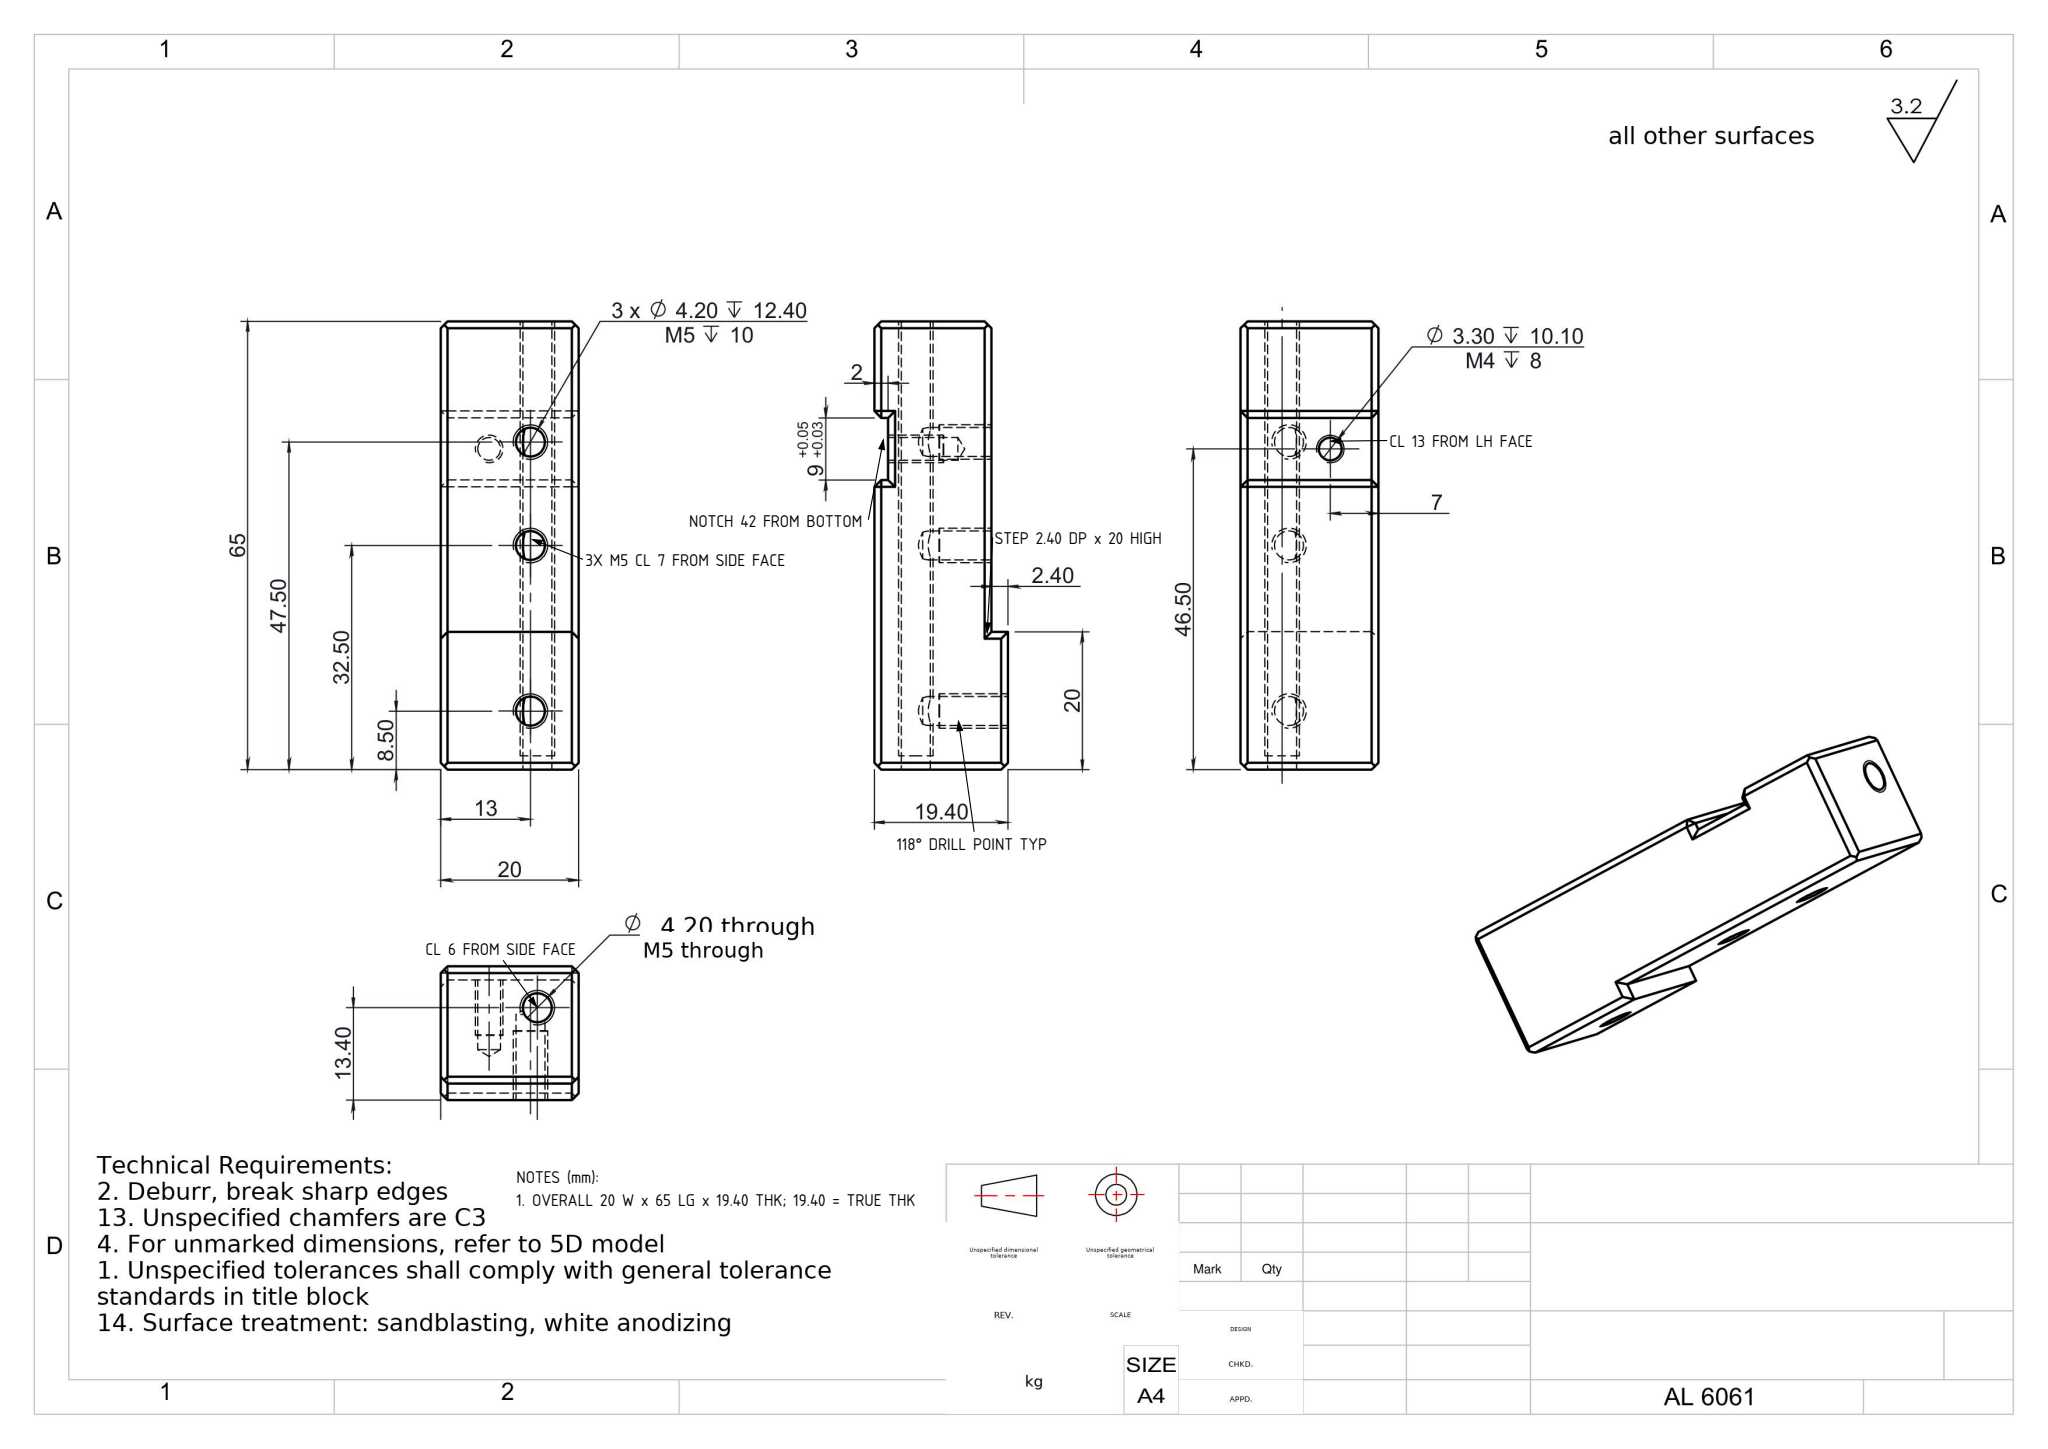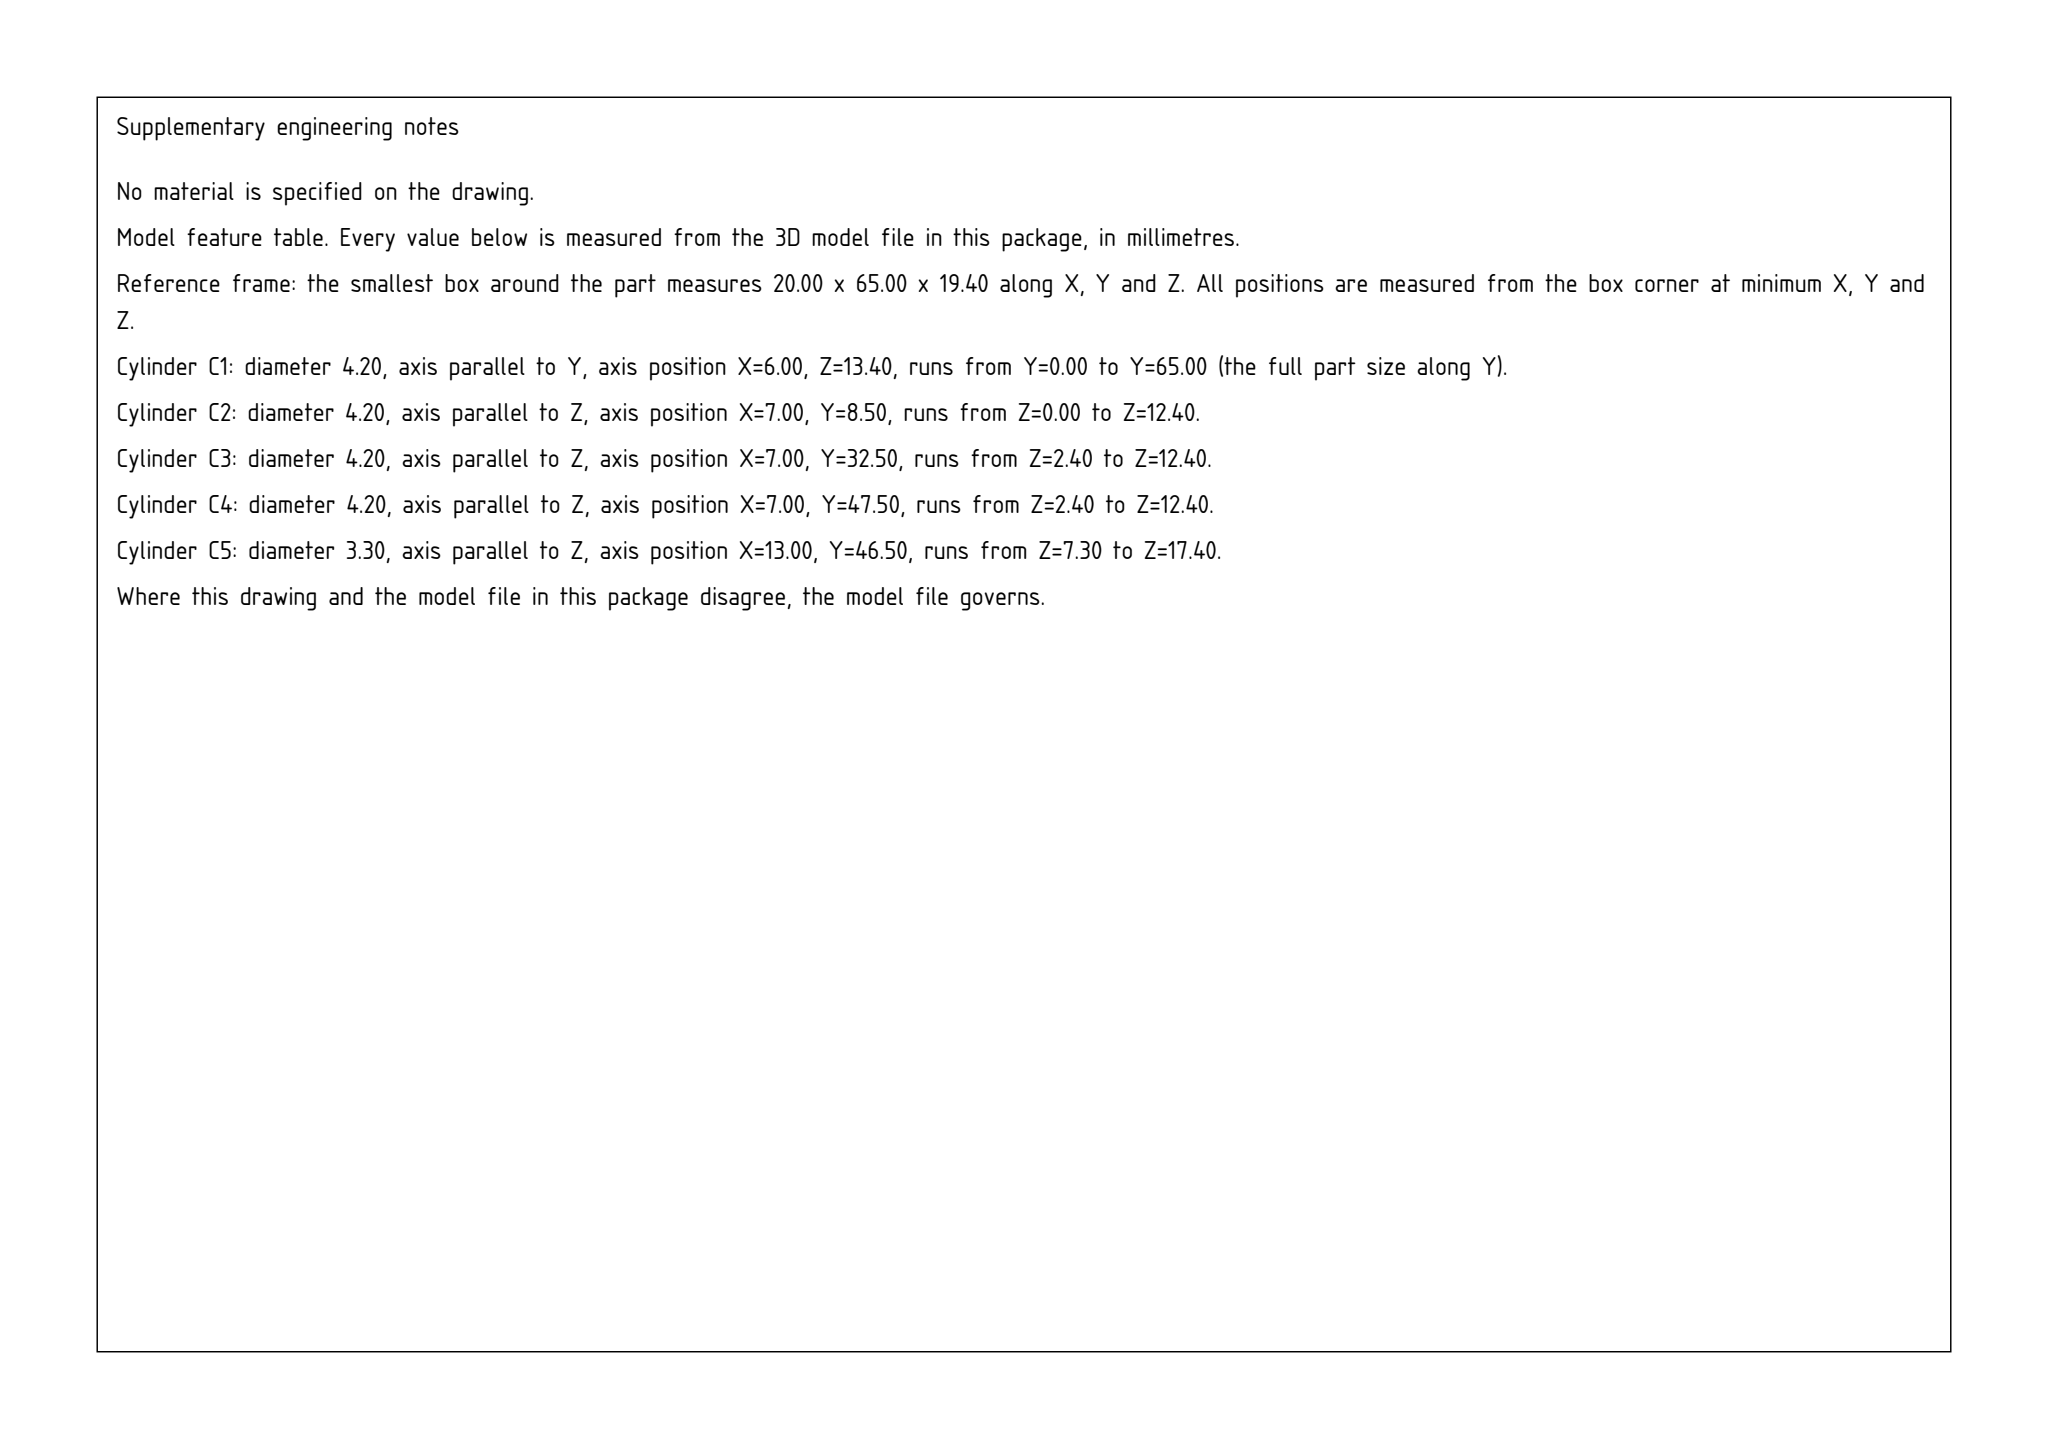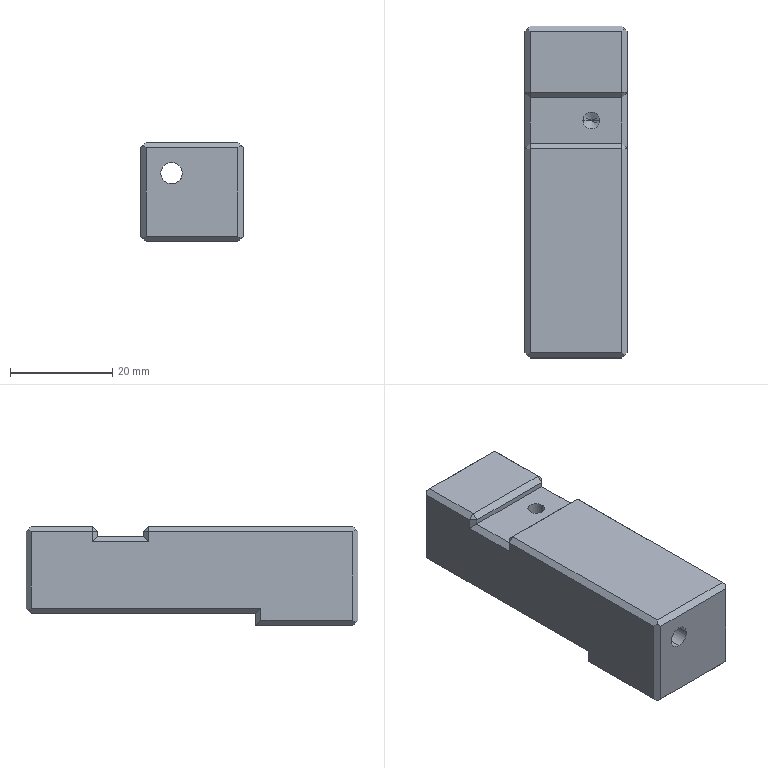Part | SolidWorks | mm | material AL 6061 | 1 solid | 57 faces | box 20 x 65 x 19.4 mm | volume 21060 mm3 | plane 42 | cylinder 10 | cone 5 | commonest cylinder face diameters 4.2 x8 3.3 x2
Drawing notes:
OVERALL 20 W x 65 LG x 19.40 THK; 19.40 = TRUE THK | from the solid: bbox_xyz [20.0, 65.0, 19.4]
2.40 DP STEP FROM BOTTOM FACE, 20 HIGH, FULL 20 WIDTH | from the solid: z-planes 0.0 & 2.4; y-plane 20.0 from y=0 bottom; bbox x=20
SIDE NOTCH 9 (+0.05/+0.03) W x 2 DP: 42 FROM BOTTOM, 14 FROM TOP | from the solid: y-planes 42.0 & 51.0 (9 wide); z-planes 17.4 & 19.4 (2 deep); bbox y=65
3x Ø4.20 DP 12.40 / M5 DP 10: CL 7 FROM SIDE FACE | from the solid: cyls dia 4.2 axis z at x=7.0, y=8.5/32.5/47.5; depths 12.4 & 10.0
Ø4.20 THRU / M5 THRU: CL 6 FROM SIDE FACE, THRU 65 | from the solid: cyl dia 4.2 axis y at [x=6.0, z=13.4], length 65 = full bbox y
Ø3.30 DP 10.10 / M4 DP 8: CL 13 FROM LH FACE (7 FROM RH FACE) | from the solid: cyl dia 3.3 axis z at [13.0, 46.5], bbox x=20 so 20-13=7; depth 10.1
DRILL POINT 118° TYP AT ALL Ø4.20 AND Ø3.30 BLIND HOLE BOTTOMS | from the solid: cones [118.0, 3.3] x2 and [118.0, 4.2] x3
build123d program:
from build123d import *

# Parameters (mm, degrees)
SKETCH1_W             = 20
SKETCH1_H             = 65
BOSS_EXTRUDE1_DEPTH   = 17
SKETCH2_W             = 20
SKETCH2_H             = 9
CUT_EXTRUDE1_DEPTH    = 2
SKETCH9_W             = 20
SKETCH9_H             = 20
BOSS_EXTRUDE2_DEPTH   = 2.4
M5_TAPPED_HOLE1_D     = 4.2
M5_TAPPED_HOLE1_DEPTH = 12.4
M5_TAPPED_HOLE1_TIP   = 1.262
M5_TAPPED_HOLE2_D     = 4.2
CHAMFER1_SIZE         = 1
CHAMFER2_SIZE         = 1
M4_TAPPED_HOLE1_D     = 3.3
M4_TAPPED_HOLE1_DEPTH = 10.1
M4_TAPPED_HOLE1_TIP   = 0.9914


with BuildPart() as part:
    # Sketch1 → Boss-Extrude1 (new body)
    with BuildSketch(Plane.XY):
        Rectangle(SKETCH1_W, SKETCH1_H)
    extrude(amount=BOSS_EXTRUDE1_DEPTH)

    # Sketch2 → Cut-Extrude1 (cut)
    with BuildSketch(Plane.XY.offset(17)):
        with Locations((0, 14)):
            Rectangle(SKETCH2_W, SKETCH2_H)
    extrude(amount=-CUT_EXTRUDE1_DEPTH, mode=Mode.SUBTRACT)

    # Sketch9 → Boss-Extrude2 (add)
    with BuildSketch(Plane(origin=(0, 0, 0), x_dir=(-1, 0, 0), z_dir=(0, 0, -1))):
        with Locations((0, -22.5)):
            Rectangle(SKETCH9_W, SKETCH9_H)
    extrude(amount=BOSS_EXTRUDE2_DEPTH)

    # M5 Tapped Hole1
    with Locations(Plane(origin=(0, 0, -2.4), x_dir=(-1, 0, 0), z_dir=(0, 0, -1))):
        with Locations((3, 0), (3, 15), (3, -24)):
            Hole(M5_TAPPED_HOLE1_D / 2, depth=M5_TAPPED_HOLE1_DEPTH)
            with Locations((0, 0, -(M5_TAPPED_HOLE1_DEPTH + M5_TAPPED_HOLE1_TIP / 2))):  # 118° drill point
                Cone(0, M5_TAPPED_HOLE1_D / 2, M5_TAPPED_HOLE1_TIP, mode=Mode.SUBTRACT)

    # M5 Tapped Hole2 (through all)
    with Locations(Plane(origin=(0, 32.5, 0), x_dir=(1, 0, 0), z_dir=(0, 1, 0))):
        with Locations((-4, -11)):
            Hole(M5_TAPPED_HOLE2_D / 2)

    # Chamfer1
    chamfer1_edges = [part.edges().sort_by_distance(p)[0] for p in [
        (-10, 25.5, 17),
        (10, 25.5, 17),
        (-10, -11.5, 17),
        (-10, 14, 15),
        (-10, 9.5, 16),
        (-10, 18.5, 16),
        (10, 14, 15),
        (10, 18.5, 16),
        (10, 9.5, 16),
        (0, 9.5, 17),
        (0, 18.5, 17),
        (10, 10, 0),
        (10, -12.5, -1.2),
        (-10, -12.5, -1.2),
        (10, -22.5, -2.4),
        (-10, -22.5, -2.4),
        (10, -11.5, 17),
        (-10, 10, 0),
        (10, -32.5, 7.3),
        (-10, -32.5, 7.3),
        (-10, 32.5, 8.5),
        (10, 32.5, 8.5),
    ]]
    chamfer(chamfer1_edges, length=CHAMFER1_SIZE)

    # Chamfer2
    chamfer2_edges = [part.edges().sort_by_distance(p)[0] for p in [
        (0, -32.5, 17),
        (0, -32.5, -2.4),
        (0, 32.5, 0),
        (0, 32.5, 17),
    ]]
    chamfer(chamfer2_edges, length=CHAMFER2_SIZE)

    # M4 Tapped Hole1
    with Locations(Plane.XY.offset(15)):
        with Locations((3, 14)):
            Hole(M4_TAPPED_HOLE1_D / 2, depth=M4_TAPPED_HOLE1_DEPTH)
            with Locations((0, 0, -(M4_TAPPED_HOLE1_DEPTH + M4_TAPPED_HOLE1_TIP / 2))):  # 118° drill point
                Cone(0, M4_TAPPED_HOLE1_D / 2, M4_TAPPED_HOLE1_TIP, mode=Mode.SUBTRACT)


solid = part.part